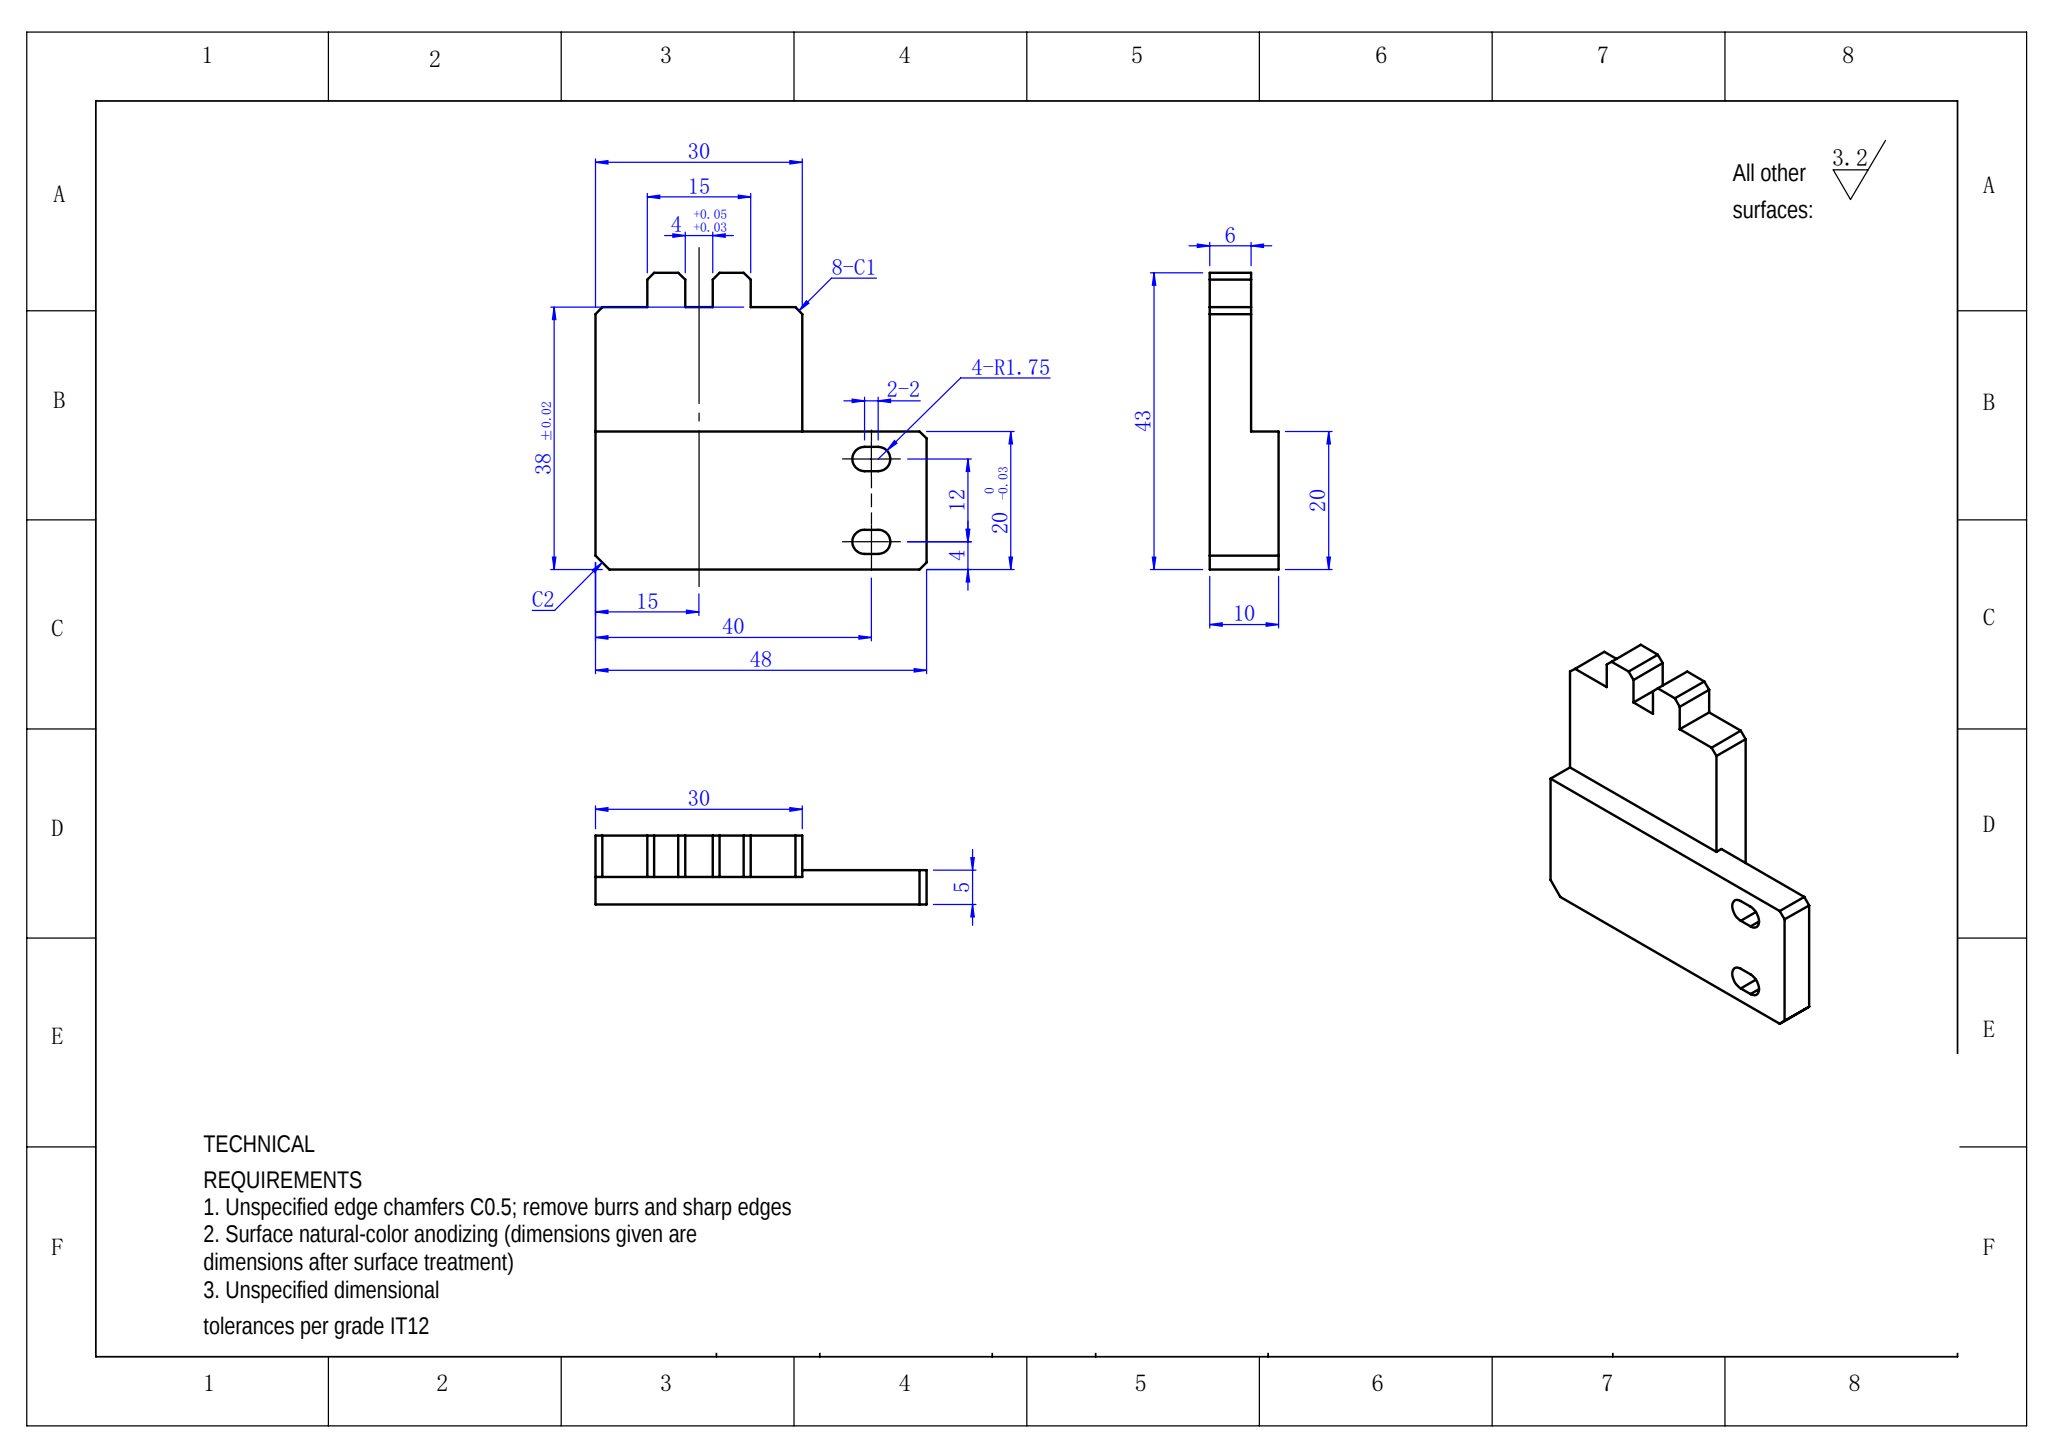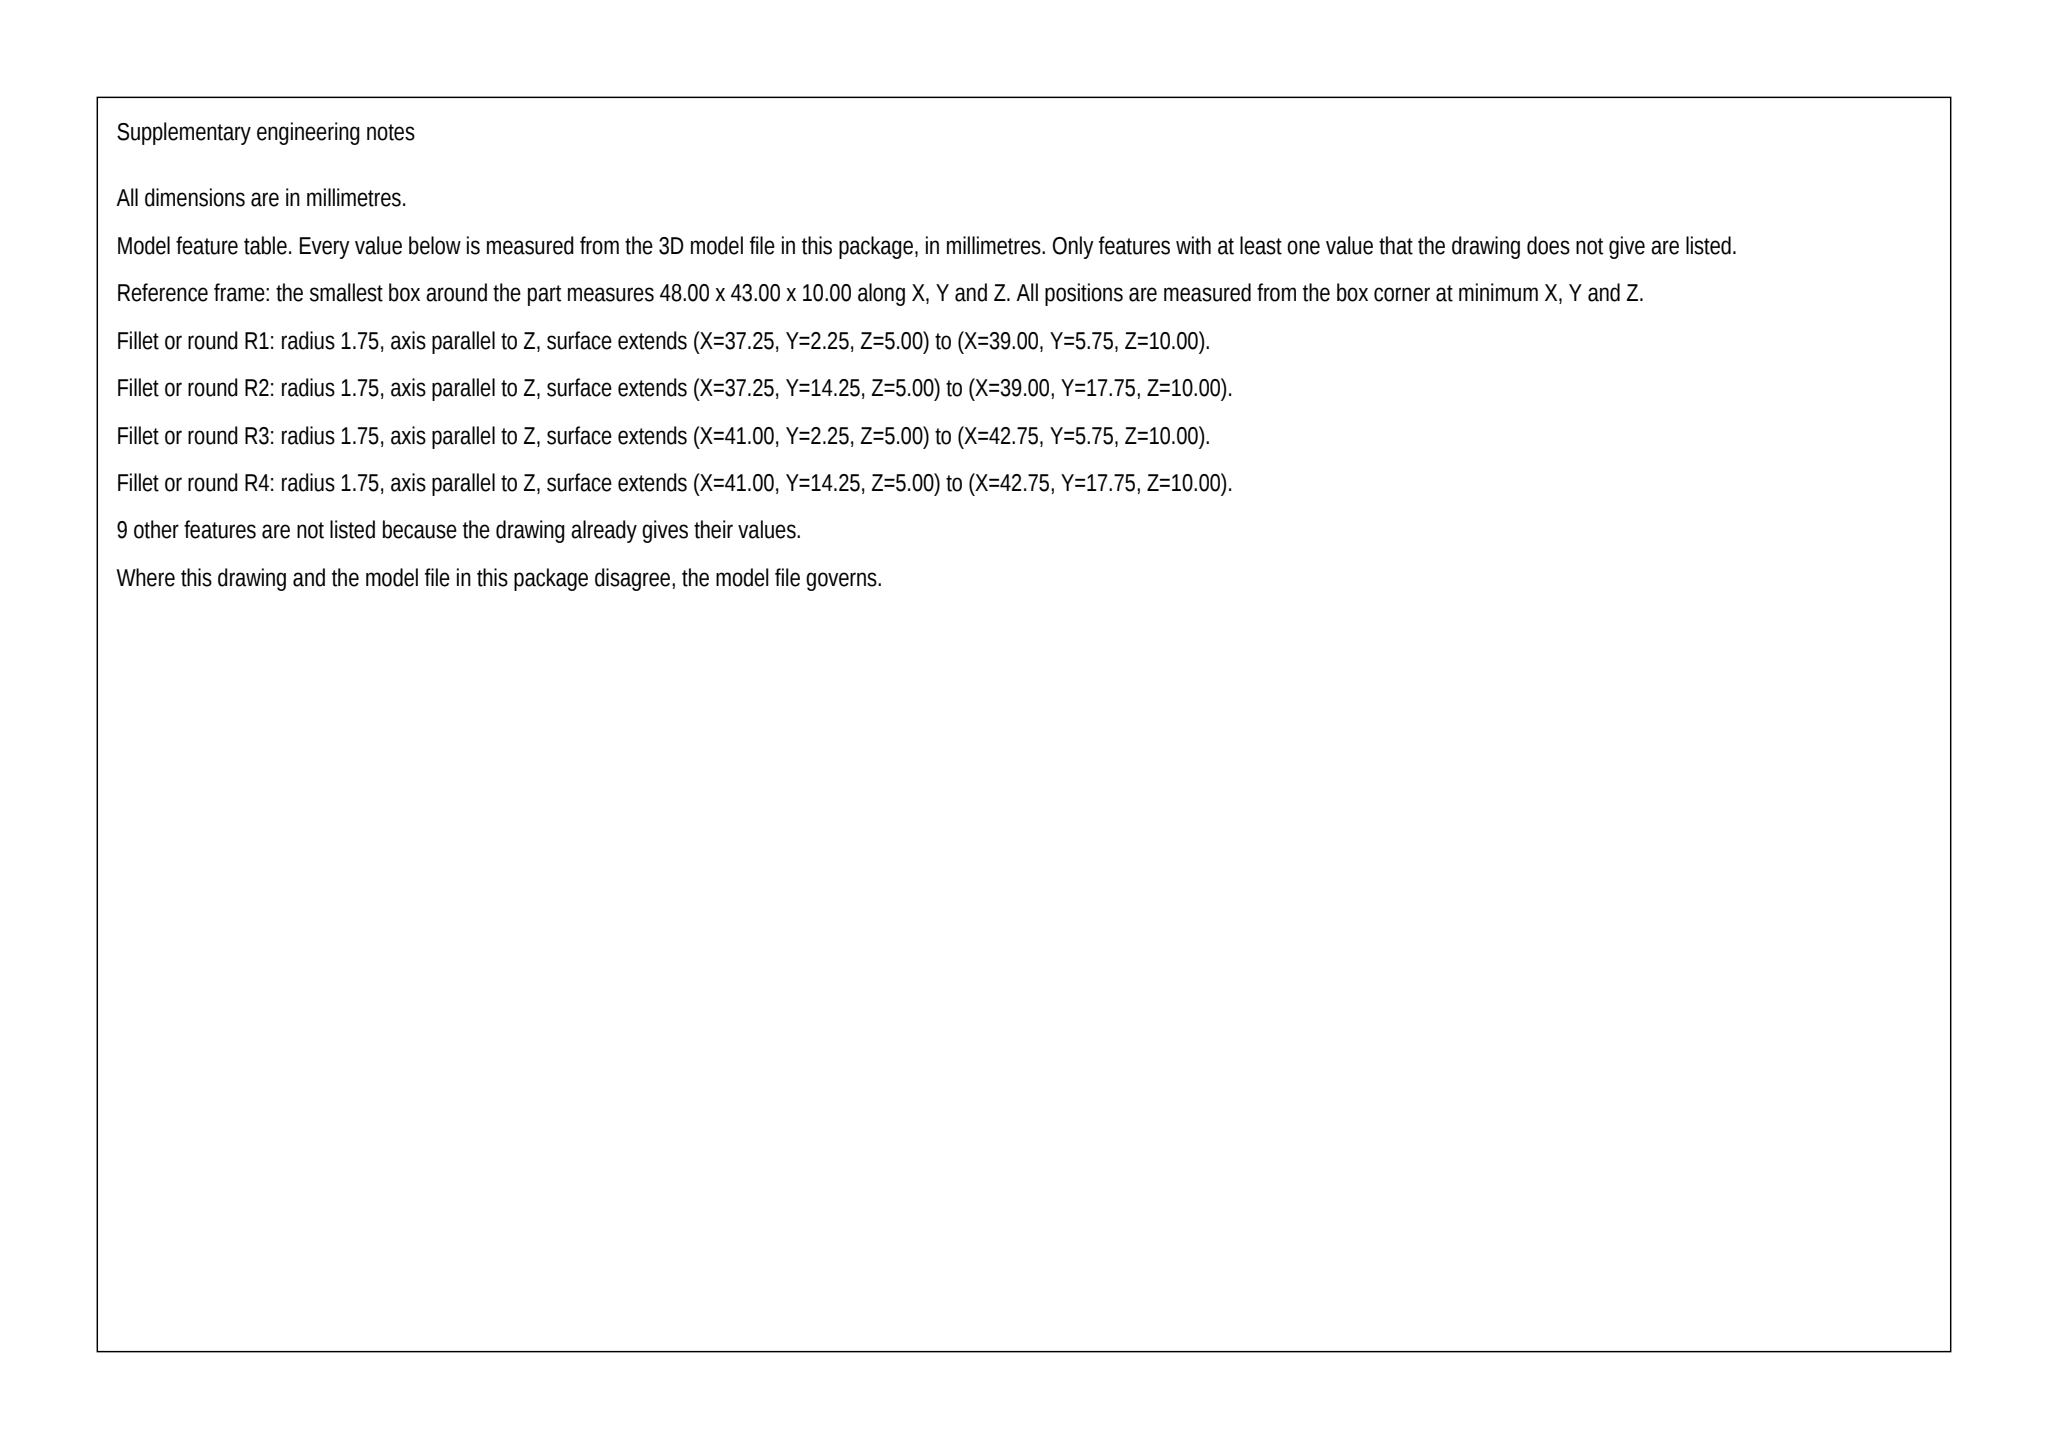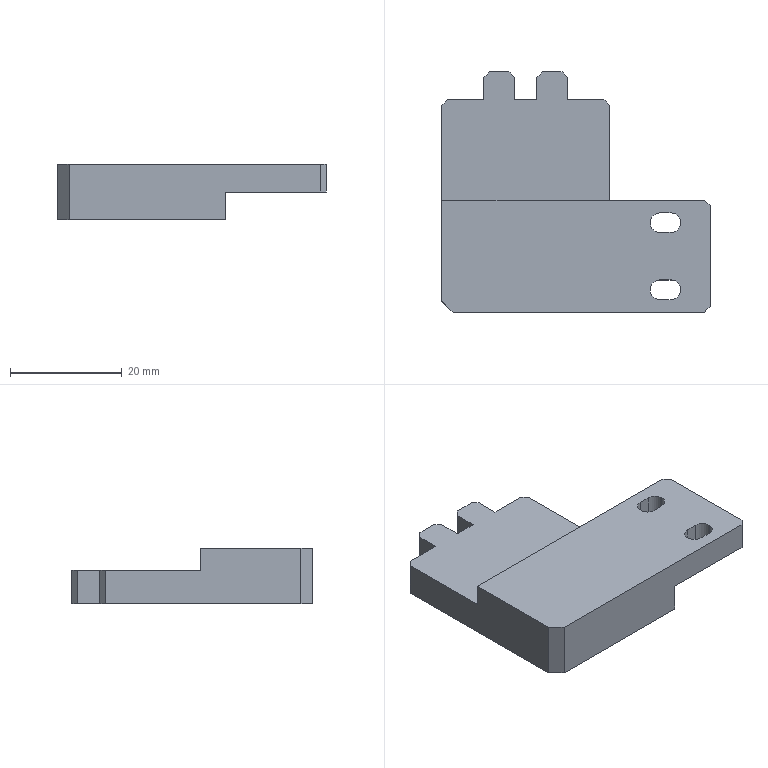Part | SolidWorks | mm | 1 solid | 37 faces | box 48 x 43 x 10 mm | volume 11161 mm3 | plane 31 | cylinder 6 | commonest cylinder face diameters 3.5 x6
build123d program:
from build123d import *

# Parameters (mm, degrees)
BOSS_EXTRUDE1_DEPTH      = 10
SKETCH2_W                = 18
SKETCH2_H                = 20
CUT_EXTRUDE1_DEPTH       = 5
SKETCH3_W                = 7.5
SKETCH3_H                = 5
SKETCH3_W_2              = 4
CUT_EXTRUDE2_DEPTH       = 66.215
SKETCH6_W                = 30
SKETCH6_H                = 23
CUT_EXTRUDE4_DEPTH       = 4
CHAMFER1_SIZE            = 1
CHAMFER2_SIZE            = 2
CHAMFER1_OF_MIRROR1_SIZE = 1
CHAMFER2_OF_MIRROR1_SIZE = 2
SKETCH4_W                = 48
SKETCH4_H                = 43
CUT_EXTRUDE3_DEPTH       = 66.215


with BuildPart() as part:
    # Sketch1 → Boss-Extrude1 (new body)
    with BuildSketch(Plane.XY):
        Polygon((0, 0), (48, 0), (48, 43), (18, 43), (18, 20), (0, 20), align=None)
    boss_extrude1 = extrude(amount=BOSS_EXTRUDE1_DEPTH)

    # Sketch2 → Cut-Extrude1 (cut)
    with BuildSketch(Plane(origin=(0, 0, 0), x_dir=(-1, 0, 0), z_dir=(0, 0, -1))):
        with Locations((-9, 10)):
            Rectangle(SKETCH2_W, SKETCH2_H)
    cut_extrude1 = extrude(amount=-CUT_EXTRUDE1_DEPTH, mode=Mode.SUBTRACT)

    # Sketch3 → Cut-Extrude2 (cut, through all)
    with BuildSketch(Plane.XY.offset(10)):
        with BuildLine():
            Line((7, 17.75), (9, 17.75))
            ThreePointArc((9, 17.75), (10.75, 16), (9, 14.25))
            Line((9, 14.25), (7, 14.25))
            ThreePointArc((7, 14.25), (5.25, 16), (7, 17.75))
        make_face()
        with BuildLine():
            Line((7, 5.75), (9, 5.75))
            ThreePointArc((9, 5.75), (10.75, 4), (9, 2.25))
            Line((9, 2.25), (7, 2.25))
            ThreePointArc((7, 2.25), (5.25, 4), (7, 5.75))
        make_face()
        with Locations((44.25, 40.5)):
            Rectangle(SKETCH3_W, SKETCH3_H)
        with Locations((33, 40.5)):
            Rectangle(SKETCH3_W_2, SKETCH3_H)
        with Locations((21.75, 40.5)):
            Rectangle(SKETCH3_W, SKETCH3_H)
    cut_extrude2 = extrude(amount=-CUT_EXTRUDE2_DEPTH, mode=Mode.SUBTRACT)

    # Sketch6 → Cut-Extrude4 (cut)
    with BuildSketch(Plane.XY.offset(10)):
        with Locations((33, 31.5)):
            Rectangle(SKETCH6_W, SKETCH6_H)
    cut_extrude4 = extrude(amount=-CUT_EXTRUDE4_DEPTH, mode=Mode.SUBTRACT)

    # Chamfer1
    chamfer1_edges = [part.edges().sort_by_distance(p)[0] for p in [
        (0, 20, 7.5),
        (0, 0, 7.5),
        (40.5, 43, 3),
        (48, 38, 3),
        (18, 38, 3),
        (25.5, 43, 3),
        (31, 43, 3),
        (35, 43, 3),
    ]]
    chamfer(chamfer1_edges, length=CHAMFER1_SIZE)

    # Chamfer2
    chamfer2_edges = [part.edges().sort_by_distance(p)[0] for p in [
        (48, 0, 5),
    ]]
    chamfer(chamfer2_edges, length=CHAMFER2_SIZE)


with BuildPart() as mirror1_1:
    # Mirror1: Boss-Extrude1 across plane
    add(boss_extrude1.mirror(Plane(origin=(0, 0, 0), x_dir=(0, 0, 1), z_dir=(1, 0, 0))))

    # Mirror1 2: Cut-Extrude1, Cut-Extrude2, Cut-Extrude4 across plane
    add(cut_extrude1.mirror(Plane(origin=(0, 0, 0), x_dir=(0, 0, 1), z_dir=(1, 0, 0))), mode=Mode.SUBTRACT)
    add(cut_extrude2.mirror(Plane(origin=(0, 0, 0), x_dir=(0, 0, 1), z_dir=(1, 0, 0))), mode=Mode.SUBTRACT)
    add(cut_extrude4.mirror(Plane(origin=(0, 0, 0), x_dir=(0, 0, 1), z_dir=(1, 0, 0))), mode=Mode.SUBTRACT)

    # Chamfer1 of Mirror1
    chamfer1_of_mirror1_edges = [mirror1_1.edges().sort_by_distance(p)[0] for p in [
        (0, 20, 7.5),
        (0, 0, 7.5),
        (-40.5, 43, 3),
        (-48, 38, 3),
        (-18, 38, 3),
        (-25.5, 43, 3),
        (-31, 43, 3),
        (-35, 43, 3),
    ]]
    chamfer(chamfer1_of_mirror1_edges, length=CHAMFER1_OF_MIRROR1_SIZE)

    # Chamfer2 of Mirror1
    chamfer2_of_mirror1_edges = [mirror1_1.edges().sort_by_distance(p)[0] for p in [
        (-48, 0, 5),
    ]]
    chamfer(chamfer2_of_mirror1_edges, length=CHAMFER2_OF_MIRROR1_SIZE)


with BuildPart() as part_1:
    add(part.part)

    # Mirror1 united with what the copies touc: union Mirror1_1
    add(mirror1_1.part)

    # Sketch4 → Cut-Extrude3 (cut, through all)
    with BuildSketch(Plane.XY.offset(10)):
        with Locations((24, 21.5)):
            Rectangle(SKETCH4_W, SKETCH4_H)
    extrude(amount=-CUT_EXTRUDE3_DEPTH, mode=Mode.SUBTRACT)


solid = part_1.part